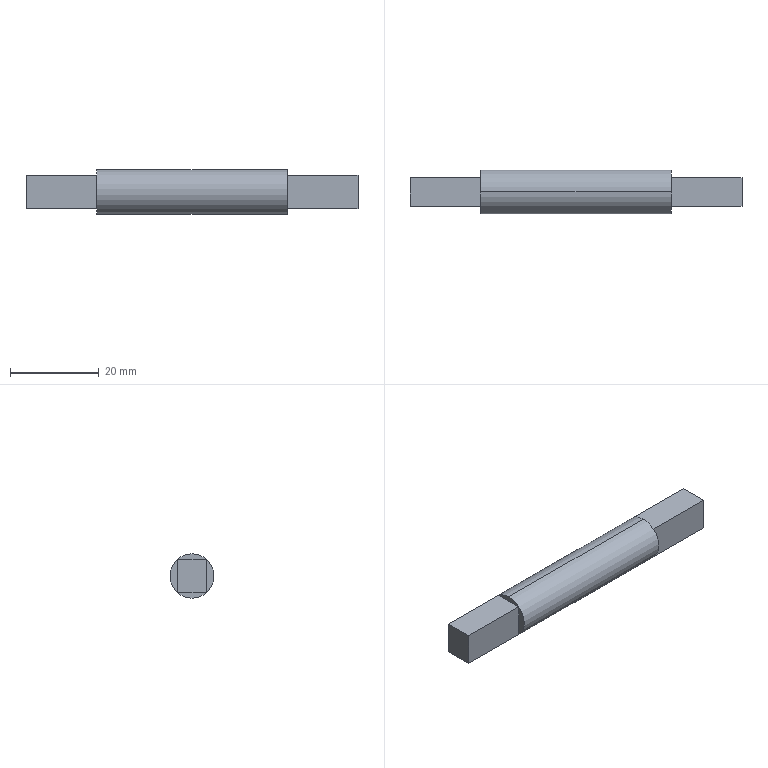Component | SolidWorks | CHEN123-AA-36-1 | 1 solid | 20 faces | box 75 x 10 x 10 mm | volume 4953 mm3 | plane 18 | cylinder 2 | commonest cylinder face diameters 10 x2
build123d program:
from build123d import *

# Parameters (mm, degrees)
SKETCH1_R           = 5
BOSS_EXTRUDE1_DEPTH = 75
SKETCH3_R           = 7.619
SKETCH3_W           = 7.664
SKETCH3_H           = 6.424
CUT_EXTRUDE2_DEPTH  = 16
SKETCH4_R           = 7.619
SKETCH4_W           = 7.664
SKETCH4_H           = 6.424
CUT_EXTRUDE3_DEPTH  = 16


with BuildPart() as part:
    # Sketch1 → Boss-Extrude1 (new body)
    with BuildSketch(Plane.XY):
        Circle(SKETCH1_R)
    extrude(amount=BOSS_EXTRUDE1_DEPTH)

    # Sketch3 → Cut-Extrude2 (cut)
    with BuildSketch(Plane.XY.offset(75)):
        Circle(SKETCH3_R)
        Rectangle(SKETCH3_W, SKETCH3_H, mode=Mode.SUBTRACT)
    extrude(amount=-CUT_EXTRUDE2_DEPTH, mode=Mode.SUBTRACT)

    # Sketch4 → Cut-Extrude3 (cut)
    with BuildSketch(Plane(origin=(0, 0, 0), x_dir=(-1, 0, 0), z_dir=(0, 0, -1))):
        Circle(SKETCH4_R)
        Rectangle(SKETCH4_W, SKETCH4_H, mode=Mode.SUBTRACT)
    extrude(amount=-CUT_EXTRUDE3_DEPTH, mode=Mode.SUBTRACT)


solid = part.part

# Placed as in the assembly
solid = solid.moved(Location((-37.501, -45.999, -172), (0, 90, 0)))
STEP:
#1=COLOUR_RGB('',0.7922,0.8196,0.9333);
#2=FILL_AREA_STYLE_COLOUR('',#1);
#3=FILL_AREA_STYLE('',(#2));
#4=SURFACE_STYLE_FILL_AREA(#3);
#5=SURFACE_SIDE_STYLE('',(#4));
#6=SURFACE_STYLE_USAGE(.BOTH.,#5);
#7=PRESENTATION_STYLE_ASSIGNMENT((#6));
#8=CARTESIAN_POINT('',(-0.8465,-1.811,-6.575));
#9=VERTEX_POINT('',#8);
#10=CARTESIAN_POINT('',(-0.8465,-1.685,-6.621));
#11=VERTEX_POINT('',#10);
#12=CARTESIAN_POINT('',(-0.8465,-1.811,-6.772));
#13=DIRECTION('',(-1.,0.,0.));
#14=DIRECTION('',(0.,0.,1.));
#15=AXIS2_PLACEMENT_3D('',#12,#13,#14);
#16=CIRCLE('',#15,0.1969);
#17=EDGE_CURVE('',#9,#11,#16,.T.);
#18=ORIENTED_EDGE('',*,*,#17,.F.);
#19=CARTESIAN_POINT('',(0.8464,-1.811,-6.575));
#20=VERTEX_POINT('',#19);
#21=CARTESIAN_POINT('',(-1.476,-1.811,-6.575));
#22=DIRECTION('',(1.,-0.,0.));
#23=VECTOR('',#22,39.37);
#24=LINE('',#21,#23);
#25=EDGE_CURVE('',#9,#20,#24,.T.);
#26=ORIENTED_EDGE('',*,*,#25,.T.);
#27=CARTESIAN_POINT('',(0.8464,-1.685,-6.621));
#28=VERTEX_POINT('',#27);
#29=CARTESIAN_POINT('',(0.8464,-1.811,-6.772));
#30=DIRECTION('',(1.,-0.,0.));
#31=DIRECTION('',(0.,0.,-1.));
#32=AXIS2_PLACEMENT_3D('',#29,#30,#31);
#33=CIRCLE('',#32,0.1969);
#34=EDGE_CURVE('',#28,#20,#33,.T.);
#35=ORIENTED_EDGE('',*,*,#34,.F.);
#36=CARTESIAN_POINT('',(0.8464,-1.685,-6.923));
#37=VERTEX_POINT('',#36);
#38=CARTESIAN_POINT('',(0.8464,-1.811,-6.772));
#39=DIRECTION('',(1.,-0.,0.));
#40=DIRECTION('',(0.,0.,-1.));
#41=AXIS2_PLACEMENT_3D('',#38,#39,#40);
#42=CIRCLE('',#41,0.1969);
#43=EDGE_CURVE('',#37,#28,#42,.T.);
#44=ORIENTED_EDGE('',*,*,#43,.F.);
#45=CARTESIAN_POINT('',(0.8464,-1.811,-6.969));
#46=VERTEX_POINT('',#45);
#47=CARTESIAN_POINT('',(0.8464,-1.811,-6.772));
#48=DIRECTION('',(1.,-0.,0.));
#49=DIRECTION('',(0.,0.,-1.));
#50=AXIS2_PLACEMENT_3D('',#47,#48,#49);
#51=CIRCLE('',#50,0.1969);
#52=EDGE_CURVE('',#46,#37,#51,.T.);
#53=ORIENTED_EDGE('',*,*,#52,.F.);
#54=CARTESIAN_POINT('',(-0.8465,-1.811,-6.969));
#55=VERTEX_POINT('',#54);
#56=CARTESIAN_POINT('',(-1.476,-1.811,-6.969));
#57=DIRECTION('',(1.,-0.,0.));
#58=VECTOR('',#57,39.37);
#59=LINE('',#56,#58);
#60=EDGE_CURVE('',#55,#46,#59,.T.);
#61=ORIENTED_EDGE('',*,*,#60,.F.);
#62=CARTESIAN_POINT('',(-0.8465,-1.685,-6.923));
#63=VERTEX_POINT('',#62);
#64=CARTESIAN_POINT('',(-0.8465,-1.811,-6.772));
#65=DIRECTION('',(-1.,0.,0.));
#66=DIRECTION('',(0.,0.,1.));
#67=AXIS2_PLACEMENT_3D('',#64,#65,#66);
#68=CIRCLE('',#67,0.1969);
#69=EDGE_CURVE('',#63,#55,#68,.T.);
#70=ORIENTED_EDGE('',*,*,#69,.F.);
#71=CARTESIAN_POINT('',(-0.8465,-1.811,-6.772));
#72=DIRECTION('',(-1.,0.,0.));
#73=DIRECTION('',(0.,0.,1.));
#74=AXIS2_PLACEMENT_3D('',#71,#72,#73);
#75=CIRCLE('',#74,0.1969);
#76=EDGE_CURVE('',#11,#63,#75,.T.);
#77=ORIENTED_EDGE('',*,*,#76,.F.);
#78=EDGE_LOOP('',(#18,#26,#35,#44,#53,#61,#70,#77));
#79=FACE_OUTER_BOUND('',#78,.T.);
#80=CARTESIAN_POINT('',(-1.476,-1.811,-6.772));
#81=DIRECTION('',(1.,-0.,0.));
#82=DIRECTION('',(0.,0.,-1.));
#83=AXIS2_PLACEMENT_3D('',#80,#81,#82);
#84=CYLINDRICAL_SURFACE('',#83,0.1969);
#85=ADVANCED_FACE('',(#79),#84,.T.);
#86=ORIENTED_EDGE('',*,*,#25,.F.);
#87=CARTESIAN_POINT('',(-0.8465,-1.937,-6.621));
#88=VERTEX_POINT('',#87);
#89=CARTESIAN_POINT('',(-0.8465,-1.811,-6.772));
#90=DIRECTION('',(-1.,0.,0.));
#91=DIRECTION('',(0.,0.,1.));
#92=AXIS2_PLACEMENT_3D('',#89,#90,#91);
#93=CIRCLE('',#92,0.1969);
#94=EDGE_CURVE('',#88,#9,#93,.T.);
#95=ORIENTED_EDGE('',*,*,#94,.F.);
#96=CARTESIAN_POINT('',(-0.8465,-1.937,-6.923));
#97=VERTEX_POINT('',#96);
#98=CARTESIAN_POINT('',(-0.8465,-1.811,-6.772));
#99=DIRECTION('',(-1.,0.,0.));
#100=DIRECTION('',(0.,0.,1.));
#101=AXIS2_PLACEMENT_3D('',#98,#99,#100);
#102=CIRCLE('',#101,0.1969);
#103=EDGE_CURVE('',#97,#88,#102,.T.);
#104=ORIENTED_EDGE('',*,*,#103,.F.);
#105=CARTESIAN_POINT('',(-0.8465,-1.811,-6.772));
#106=DIRECTION('',(-1.,0.,0.));
#107=DIRECTION('',(0.,0.,1.));
#108=AXIS2_PLACEMENT_3D('',#105,#106,#107);
#109=CIRCLE('',#108,0.1969);
#110=EDGE_CURVE('',#55,#97,#109,.T.);
#111=ORIENTED_EDGE('',*,*,#110,.F.);
#112=ORIENTED_EDGE('',*,*,#60,.T.);
#113=CARTESIAN_POINT('',(0.8464,-1.937,-6.923));
#114=VERTEX_POINT('',#113);
#115=CARTESIAN_POINT('',(0.8464,-1.811,-6.772));
#116=DIRECTION('',(1.,-0.,0.));
#117=DIRECTION('',(0.,0.,-1.));
#118=AXIS2_PLACEMENT_3D('',#115,#116,#117);
#119=CIRCLE('',#118,0.1969);
#120=EDGE_CURVE('',#114,#46,#119,.T.);
#121=ORIENTED_EDGE('',*,*,#120,.F.);
#122=CARTESIAN_POINT('',(0.8464,-1.937,-6.621));
#123=VERTEX_POINT('',#122);
#124=CARTESIAN_POINT('',(0.8464,-1.811,-6.772));
#125=DIRECTION('',(1.,-0.,0.));
#126=DIRECTION('',(0.,0.,-1.));
#127=AXIS2_PLACEMENT_3D('',#124,#125,#126);
#128=CIRCLE('',#127,0.1969);
#129=EDGE_CURVE('',#123,#114,#128,.T.);
#130=ORIENTED_EDGE('',*,*,#129,.F.);
#131=CARTESIAN_POINT('',(0.8464,-1.811,-6.772));
#132=DIRECTION('',(1.,-0.,0.));
#133=DIRECTION('',(0.,0.,-1.));
#134=AXIS2_PLACEMENT_3D('',#131,#132,#133);
#135=CIRCLE('',#134,0.1969);
#136=EDGE_CURVE('',#20,#123,#135,.T.);
#137=ORIENTED_EDGE('',*,*,#136,.F.);
#138=EDGE_LOOP('',(#86,#95,#104,#111,#112,#121,#130,#137));
#139=FACE_OUTER_BOUND('',#138,.T.);
#140=CARTESIAN_POINT('',(-1.476,-1.811,-6.772));
#141=DIRECTION('',(1.,-0.,0.));
#142=DIRECTION('',(0.,0.,-1.));
#143=AXIS2_PLACEMENT_3D('',#140,#141,#142);
#144=CYLINDRICAL_SURFACE('',#143,0.1969);
#145=ADVANCED_FACE('',(#139),#144,.T.);
#146=ORIENTED_EDGE('',*,*,#76,.T.);
#147=CARTESIAN_POINT('',(-0.8465,-1.685,-6.923));
#148=DIRECTION('',(-0.,-0.,-1.));
#149=VECTOR('',#148,39.37);
#150=LINE('',#147,#149);
#151=EDGE_CURVE('',#11,#63,#150,.T.);
#152=ORIENTED_EDGE('',*,*,#151,.F.);
#153=EDGE_LOOP('',(#146,#152));
#154=FACE_OUTER_BOUND('',#153,.T.);
#155=CARTESIAN_POINT('',(-0.8465,-1.811,-6.772));
#156=DIRECTION('',(-1.,0.,0.));
#157=DIRECTION('',(0.,0.,1.));
#158=AXIS2_PLACEMENT_3D('',#155,#156,#157);
#159=PLANE('',#158);
#160=ADVANCED_FACE('',(#154),#159,.T.);
#161=ORIENTED_EDGE('',*,*,#69,.T.);
#162=ORIENTED_EDGE('',*,*,#110,.T.);
#163=CARTESIAN_POINT('',(-0.8465,-1.685,-6.923));
#164=DIRECTION('',(-0.,-1.,0.));
#165=VECTOR('',#164,39.37);
#166=LINE('',#163,#165);
#167=EDGE_CURVE('',#63,#97,#166,.T.);
#168=ORIENTED_EDGE('',*,*,#167,.F.);
#169=EDGE_LOOP('',(#161,#162,#168));
#170=FACE_OUTER_BOUND('',#169,.T.);
#171=CARTESIAN_POINT('',(-0.8465,-1.811,-6.772));
#172=DIRECTION('',(-1.,0.,0.));
#173=DIRECTION('',(0.,0.,1.));
#174=AXIS2_PLACEMENT_3D('',#171,#172,#173);
#175=PLANE('',#174);
#176=ADVANCED_FACE('',(#170),#175,.T.);
#177=ORIENTED_EDGE('',*,*,#103,.T.);
#178=CARTESIAN_POINT('',(-0.8465,-1.937,-6.923));
#179=DIRECTION('',(0.,0.,1.));
#180=VECTOR('',#179,39.37);
#181=LINE('',#178,#180);
#182=EDGE_CURVE('',#97,#88,#181,.T.);
#183=ORIENTED_EDGE('',*,*,#182,.F.);
#184=EDGE_LOOP('',(#177,#183));
#185=FACE_OUTER_BOUND('',#184,.T.);
#186=CARTESIAN_POINT('',(-0.8465,-1.811,-6.772));
#187=DIRECTION('',(-1.,0.,0.));
#188=DIRECTION('',(0.,0.,1.));
#189=AXIS2_PLACEMENT_3D('',#186,#187,#188);
#190=PLANE('',#189);
#191=ADVANCED_FACE('',(#185),#190,.T.);
#192=ORIENTED_EDGE('',*,*,#94,.T.);
#193=ORIENTED_EDGE('',*,*,#17,.T.);
#194=CARTESIAN_POINT('',(-0.8465,-1.685,-6.621));
#195=DIRECTION('',(0.,1.,-0.));
#196=VECTOR('',#195,39.37);
#197=LINE('',#194,#196);
#198=EDGE_CURVE('',#88,#11,#197,.T.);
#199=ORIENTED_EDGE('',*,*,#198,.F.);
#200=EDGE_LOOP('',(#192,#193,#199));
#201=FACE_OUTER_BOUND('',#200,.T.);
#202=CARTESIAN_POINT('',(-0.8465,-1.811,-6.772));
#203=DIRECTION('',(-1.,0.,0.));
#204=DIRECTION('',(0.,0.,1.));
#205=AXIS2_PLACEMENT_3D('',#202,#203,#204);
#206=PLANE('',#205);
#207=ADVANCED_FACE('',(#201),#206,.T.);
#208=CARTESIAN_POINT('',(-1.476,-1.937,-6.621));
#209=VERTEX_POINT('',#208);
#210=CARTESIAN_POINT('',(-1.476,-1.685,-6.621));
#211=VERTEX_POINT('',#210);
#212=CARTESIAN_POINT('',(-1.476,-1.685,-6.621));
#213=DIRECTION('',(0.,1.,-0.));
#214=VECTOR('',#213,39.37);
#215=LINE('',#212,#214);
#216=EDGE_CURVE('',#209,#211,#215,.T.);
#217=ORIENTED_EDGE('',*,*,#216,.F.);
#218=CARTESIAN_POINT('',(-0.8465,-1.937,-6.621));
#219=DIRECTION('',(-1.,0.,0.));
#220=VECTOR('',#219,39.37);
#221=LINE('',#218,#220);
#222=EDGE_CURVE('',#88,#209,#221,.T.);
#223=ORIENTED_EDGE('',*,*,#222,.F.);
#224=ORIENTED_EDGE('',*,*,#198,.T.);
#225=CARTESIAN_POINT('',(-0.8465,-1.685,-6.621));
#226=DIRECTION('',(-1.,0.,0.));
#227=VECTOR('',#226,39.37);
#228=LINE('',#225,#227);
#229=EDGE_CURVE('',#11,#211,#228,.T.);
#230=ORIENTED_EDGE('',*,*,#229,.T.);
#231=EDGE_LOOP('',(#217,#223,#224,#230));
#232=FACE_OUTER_BOUND('',#231,.T.);
#233=CARTESIAN_POINT('',(-0.8465,-1.685,-6.621));
#234=DIRECTION('',(0.,0.,1.));
#235=DIRECTION('',(1.,-0.,0.));
#236=AXIS2_PLACEMENT_3D('',#233,#234,#235);
#237=PLANE('',#236);
#238=ADVANCED_FACE('',(#232),#237,.T.);
#239=CARTESIAN_POINT('',(-1.476,-1.937,-6.923));
#240=VERTEX_POINT('',#239);
#241=CARTESIAN_POINT('',(-1.476,-1.937,-6.923));
#242=DIRECTION('',(0.,0.,1.));
#243=VECTOR('',#242,39.37);
#244=LINE('',#241,#243);
#245=EDGE_CURVE('',#240,#209,#244,.T.);
#246=ORIENTED_EDGE('',*,*,#245,.F.);
#247=CARTESIAN_POINT('',(-0.8465,-1.937,-6.923));
#248=DIRECTION('',(-1.,0.,0.));
#249=VECTOR('',#248,39.37);
#250=LINE('',#247,#249);
#251=EDGE_CURVE('',#97,#240,#250,.T.);
#252=ORIENTED_EDGE('',*,*,#251,.F.);
#253=ORIENTED_EDGE('',*,*,#182,.T.);
#254=ORIENTED_EDGE('',*,*,#222,.T.);
#255=EDGE_LOOP('',(#246,#252,#253,#254));
#256=FACE_OUTER_BOUND('',#255,.T.);
#257=CARTESIAN_POINT('',(-0.8465,-1.937,-6.923));
#258=DIRECTION('',(-0.,-1.,0.));
#259=DIRECTION('',(1.,-0.,0.));
#260=AXIS2_PLACEMENT_3D('',#257,#258,#259);
#261=PLANE('',#260);
#262=ADVANCED_FACE('',(#256),#261,.T.);
#263=CARTESIAN_POINT('',(-1.476,-1.685,-6.923));
#264=VERTEX_POINT('',#263);
#265=CARTESIAN_POINT('',(-1.476,-1.685,-6.923));
#266=DIRECTION('',(-0.,-1.,0.));
#267=VECTOR('',#266,39.37);
#268=LINE('',#265,#267);
#269=EDGE_CURVE('',#264,#240,#268,.T.);
#270=ORIENTED_EDGE('',*,*,#269,.F.);
#271=CARTESIAN_POINT('',(-0.8465,-1.685,-6.923));
#272=DIRECTION('',(-1.,0.,0.));
#273=VECTOR('',#272,39.37);
#274=LINE('',#271,#273);
#275=EDGE_CURVE('',#63,#264,#274,.T.);
#276=ORIENTED_EDGE('',*,*,#275,.F.);
#277=ORIENTED_EDGE('',*,*,#167,.T.);
#278=ORIENTED_EDGE('',*,*,#251,.T.);
#279=EDGE_LOOP('',(#270,#276,#277,#278));
#280=FACE_OUTER_BOUND('',#279,.T.);
#281=CARTESIAN_POINT('',(-0.8465,-1.685,-6.923));
#282=DIRECTION('',(-0.,-0.,-1.));
#283=DIRECTION('',(-1.,0.,0.));
#284=AXIS2_PLACEMENT_3D('',#281,#282,#283);
#285=PLANE('',#284);
#286=ADVANCED_FACE('',(#280),#285,.T.);
#287=CARTESIAN_POINT('',(-1.476,-1.685,-6.923));
#288=DIRECTION('',(-0.,-0.,-1.));
#289=VECTOR('',#288,39.37);
#290=LINE('',#287,#289);
#291=EDGE_CURVE('',#211,#264,#290,.T.);
#292=ORIENTED_EDGE('',*,*,#291,.F.);
#293=ORIENTED_EDGE('',*,*,#229,.F.);
#294=ORIENTED_EDGE('',*,*,#151,.T.);
#295=ORIENTED_EDGE('',*,*,#275,.T.);
#296=EDGE_LOOP('',(#292,#293,#294,#295));
#297=FACE_OUTER_BOUND('',#296,.T.);
#298=CARTESIAN_POINT('',(-0.8465,-1.685,-6.923));
#299=DIRECTION('',(0.,1.,-0.));
#300=DIRECTION('',(-1.,0.,0.));
#301=AXIS2_PLACEMENT_3D('',#298,#299,#300);
#302=PLANE('',#301);
#303=ADVANCED_FACE('',(#297),#302,.T.);
#304=ORIENTED_EDGE('',*,*,#245,.T.);
#305=ORIENTED_EDGE('',*,*,#216,.T.);
#306=ORIENTED_EDGE('',*,*,#291,.T.);
#307=ORIENTED_EDGE('',*,*,#269,.T.);
#308=EDGE_LOOP('',(#304,#305,#306,#307));
#309=FACE_OUTER_BOUND('',#308,.T.);
#310=CARTESIAN_POINT('',(-1.476,-1.811,-6.772));
#311=DIRECTION('',(-1.,0.,0.));
#312=DIRECTION('',(0.,0.,1.));
#313=AXIS2_PLACEMENT_3D('',#310,#311,#312);
#314=PLANE('',#313);
#315=ADVANCED_FACE('',(#309),#314,.T.);
#316=ORIENTED_EDGE('',*,*,#43,.T.);
#317=CARTESIAN_POINT('',(0.8464,-1.685,-6.923));
#318=DIRECTION('',(0.,0.,1.));
#319=VECTOR('',#318,39.37);
#320=LINE('',#317,#319);
#321=EDGE_CURVE('',#37,#28,#320,.T.);
#322=ORIENTED_EDGE('',*,*,#321,.F.);
#323=EDGE_LOOP('',(#316,#322));
#324=FACE_OUTER_BOUND('',#323,.T.);
#325=CARTESIAN_POINT('',(0.8464,-1.811,-6.772));
#326=DIRECTION('',(1.,-0.,0.));
#327=DIRECTION('',(-0.,-0.,-1.));
#328=AXIS2_PLACEMENT_3D('',#325,#326,#327);
#329=PLANE('',#328);
#330=ADVANCED_FACE('',(#324),#329,.T.);
#331=ORIENTED_EDGE('',*,*,#34,.T.);
#332=ORIENTED_EDGE('',*,*,#136,.T.);
#333=CARTESIAN_POINT('',(0.8464,-1.685,-6.621));
#334=DIRECTION('',(-0.,-1.,0.));
#335=VECTOR('',#334,39.37);
#336=LINE('',#333,#335);
#337=EDGE_CURVE('',#28,#123,#336,.T.);
#338=ORIENTED_EDGE('',*,*,#337,.F.);
#339=EDGE_LOOP('',(#331,#332,#338));
#340=FACE_OUTER_BOUND('',#339,.T.);
#341=CARTESIAN_POINT('',(0.8464,-1.811,-6.772));
#342=DIRECTION('',(1.,-0.,0.));
#343=DIRECTION('',(-0.,-0.,-1.));
#344=AXIS2_PLACEMENT_3D('',#341,#342,#343);
#345=PLANE('',#344);
#346=ADVANCED_FACE('',(#340),#345,.T.);
#347=ORIENTED_EDGE('',*,*,#129,.T.);
#348=CARTESIAN_POINT('',(0.8464,-1.937,-6.621));
#349=DIRECTION('',(-0.,-0.,-1.));
#350=VECTOR('',#349,39.37);
#351=LINE('',#348,#350);
#352=EDGE_CURVE('',#123,#114,#351,.T.);
#353=ORIENTED_EDGE('',*,*,#352,.F.);
#354=EDGE_LOOP('',(#347,#353));
#355=FACE_OUTER_BOUND('',#354,.T.);
#356=CARTESIAN_POINT('',(0.8464,-1.811,-6.772));
#357=DIRECTION('',(1.,-0.,0.));
#358=DIRECTION('',(-0.,-0.,-1.));
#359=AXIS2_PLACEMENT_3D('',#356,#357,#358);
#360=PLANE('',#359);
#361=ADVANCED_FACE('',(#355),#360,.T.);
#362=ORIENTED_EDGE('',*,*,#120,.T.);
#363=ORIENTED_EDGE('',*,*,#52,.T.);
#364=CARTESIAN_POINT('',(0.8464,-1.937,-6.923));
#365=DIRECTION('',(0.,1.,-0.));
#366=VECTOR('',#365,39.37);
#367=LINE('',#364,#366);
#368=EDGE_CURVE('',#114,#37,#367,.T.);
#369=ORIENTED_EDGE('',*,*,#368,.F.);
#370=EDGE_LOOP('',(#362,#363,#369));
#371=FACE_OUTER_BOUND('',#370,.T.);
#372=CARTESIAN_POINT('',(0.8464,-1.811,-6.772));
#373=DIRECTION('',(1.,-0.,0.));
#374=DIRECTION('',(-0.,-0.,-1.));
#375=AXIS2_PLACEMENT_3D('',#372,#373,#374);
#376=PLANE('',#375);
#377=ADVANCED_FACE('',(#371),#376,.T.);
#378=CARTESIAN_POINT('',(1.476,-1.937,-6.923));
#379=VERTEX_POINT('',#378);
#380=CARTESIAN_POINT('',(1.476,-1.685,-6.923));
#381=VERTEX_POINT('',#380);
#382=CARTESIAN_POINT('',(1.476,-1.937,-6.923));
#383=DIRECTION('',(0.,1.,-0.));
#384=VECTOR('',#383,39.37);
#385=LINE('',#382,#384);
#386=EDGE_CURVE('',#379,#381,#385,.T.);
#387=ORIENTED_EDGE('',*,*,#386,.F.);
#388=CARTESIAN_POINT('',(0.8464,-1.937,-6.923));
#389=DIRECTION('',(1.,-0.,0.));
#390=VECTOR('',#389,39.37);
#391=LINE('',#388,#390);
#392=EDGE_CURVE('',#114,#379,#391,.T.);
#393=ORIENTED_EDGE('',*,*,#392,.F.);
#394=ORIENTED_EDGE('',*,*,#368,.T.);
#395=CARTESIAN_POINT('',(0.8464,-1.685,-6.923));
#396=DIRECTION('',(1.,-0.,0.));
#397=VECTOR('',#396,39.37);
#398=LINE('',#395,#397);
#399=EDGE_CURVE('',#37,#381,#398,.T.);
#400=ORIENTED_EDGE('',*,*,#399,.T.);
#401=EDGE_LOOP('',(#387,#393,#394,#400));
#402=FACE_OUTER_BOUND('',#401,.T.);
#403=CARTESIAN_POINT('',(0.8464,-1.937,-6.923));
#404=DIRECTION('',(-0.,-0.,-1.));
#405=DIRECTION('',(-1.,0.,0.));
#406=AXIS2_PLACEMENT_3D('',#403,#404,#405);
#407=PLANE('',#406);
#408=ADVANCED_FACE('',(#402),#407,.T.);
#409=CARTESIAN_POINT('',(1.476,-1.937,-6.621));
#410=VERTEX_POINT('',#409);
#411=CARTESIAN_POINT('',(1.476,-1.937,-6.621));
#412=DIRECTION('',(-0.,-0.,-1.));
#413=VECTOR('',#412,39.37);
#414=LINE('',#411,#413);
#415=EDGE_CURVE('',#410,#379,#414,.T.);
#416=ORIENTED_EDGE('',*,*,#415,.F.);
#417=CARTESIAN_POINT('',(0.8464,-1.937,-6.621));
#418=DIRECTION('',(1.,-0.,0.));
#419=VECTOR('',#418,39.37);
#420=LINE('',#417,#419);
#421=EDGE_CURVE('',#123,#410,#420,.T.);
#422=ORIENTED_EDGE('',*,*,#421,.F.);
#423=ORIENTED_EDGE('',*,*,#352,.T.);
#424=ORIENTED_EDGE('',*,*,#392,.T.);
#425=EDGE_LOOP('',(#416,#422,#423,#424));
#426=FACE_OUTER_BOUND('',#425,.T.);
#427=CARTESIAN_POINT('',(0.8464,-1.937,-6.621));
#428=DIRECTION('',(-0.,-1.,0.));
#429=DIRECTION('',(1.,-0.,0.));
#430=AXIS2_PLACEMENT_3D('',#427,#428,#429);
#431=PLANE('',#430);
#432=ADVANCED_FACE('',(#426),#431,.T.);
#433=CARTESIAN_POINT('',(1.476,-1.685,-6.621));
#434=VERTEX_POINT('',#433);
#435=CARTESIAN_POINT('',(1.476,-1.685,-6.621));
#436=DIRECTION('',(-0.,-1.,0.));
#437=VECTOR('',#436,39.37);
#438=LINE('',#435,#437);
#439=EDGE_CURVE('',#434,#410,#438,.T.);
#440=ORIENTED_EDGE('',*,*,#439,.F.);
#441=CARTESIAN_POINT('',(0.8464,-1.685,-6.621));
#442=DIRECTION('',(1.,-0.,0.));
#443=VECTOR('',#442,39.37);
#444=LINE('',#441,#443);
#445=EDGE_CURVE('',#28,#434,#444,.T.);
#446=ORIENTED_EDGE('',*,*,#445,.F.);
#447=ORIENTED_EDGE('',*,*,#337,.T.);
#448=ORIENTED_EDGE('',*,*,#421,.T.);
#449=EDGE_LOOP('',(#440,#446,#447,#448));
#450=FACE_OUTER_BOUND('',#449,.T.);
#451=CARTESIAN_POINT('',(0.8464,-1.685,-6.621));
#452=DIRECTION('',(0.,0.,1.));
#453=DIRECTION('',(1.,-0.,0.));
#454=AXIS2_PLACEMENT_3D('',#451,#452,#453);
#455=PLANE('',#454);
#456=ADVANCED_FACE('',(#450),#455,.T.);
#457=CARTESIAN_POINT('',(1.476,-1.685,-6.923));
#458=DIRECTION('',(0.,0.,1.));
#459=VECTOR('',#458,39.37);
#460=LINE('',#457,#459);
#461=EDGE_CURVE('',#381,#434,#460,.T.);
#462=ORIENTED_EDGE('',*,*,#461,.F.);
#463=ORIENTED_EDGE('',*,*,#399,.F.);
#464=ORIENTED_EDGE('',*,*,#321,.T.);
#465=ORIENTED_EDGE('',*,*,#445,.T.);
#466=EDGE_LOOP('',(#462,#463,#464,#465));
#467=FACE_OUTER_BOUND('',#466,.T.);
#468=CARTESIAN_POINT('',(0.8464,-1.685,-6.923));
#469=DIRECTION('',(0.,1.,-0.));
#470=DIRECTION('',(-1.,0.,0.));
#471=AXIS2_PLACEMENT_3D('',#468,#469,#470);
#472=PLANE('',#471);
#473=ADVANCED_FACE('',(#467),#472,.T.);
#474=ORIENTED_EDGE('',*,*,#386,.T.);
#475=ORIENTED_EDGE('',*,*,#461,.T.);
#476=ORIENTED_EDGE('',*,*,#439,.T.);
#477=ORIENTED_EDGE('',*,*,#415,.T.);
#478=EDGE_LOOP('',(#474,#475,#476,#477));
#479=FACE_OUTER_BOUND('',#478,.T.);
#480=CARTESIAN_POINT('',(1.476,-1.811,-6.772));
#481=DIRECTION('',(-1.,0.,0.));
#482=DIRECTION('',(0.,0.,1.));
#483=AXIS2_PLACEMENT_3D('',#480,#481,#482);
#484=PLANE('',#483);
#485=ADVANCED_FACE('',(#479),#484,.F.);
#486=CLOSED_SHELL('',(#85,#145,#160,#176,#191,#207,#238,#262,#286,#303,#315,#330,#346,#361,#377,#408,#432,#456,#473,#485));
#487=MANIFOLD_SOLID_BREP('',#486);
#488=STYLED_ITEM('',(#7),#487);
#489=PRESENTATION_LAYER_ASSIGNMENT('','',(#488));
#490=CARTESIAN_POINT('',(0.,0.,0.));
#491=DIRECTION('',(0.,0.,1.));
#492=DIRECTION('',(1.,0.,0.));
#493=AXIS2_PLACEMENT_3D('',#490,#491,#492);
#494=(LENGTH_UNIT()NAMED_UNIT(*)SI_UNIT($,.METRE.));
#495=LENGTH_MEASURE_WITH_UNIT(LENGTH_MEASURE(0.0254),#494);
#496=DIMENSIONAL_EXPONENTS(1.,0.,0.,0.,0.,0.,0.);
#497=(CONVERSION_BASED_UNIT('',#495)LENGTH_UNIT()NAMED_UNIT(#496));
#498=UNCERTAINTY_MEASURE_WITH_UNIT(LENGTH_MEASURE(0.00001),#497,'','');
#499=(NAMED_UNIT(*)PLANE_ANGLE_UNIT()SI_UNIT($,.RADIAN.));
#500=(NAMED_UNIT(*)SI_UNIT($,.STERADIAN.)SOLID_ANGLE_UNIT());
#501=(GEOMETRIC_REPRESENTATION_CONTEXT(3)GLOBAL_UNCERTAINTY_ASSIGNED_CONTEXT((#498))GLOBAL_UNIT_ASSIGNED_CONTEXT((#497,#499,#500))REPRESENTATION_CONTEXT('',''));
#502=ADVANCED_BREP_SHAPE_REPRESENTATION('',(#487,#493),#501);
#503=(LENGTH_UNIT()NAMED_UNIT(*)SI_UNIT($,.METRE.));
#504=LENGTH_MEASURE_WITH_UNIT(LENGTH_MEASURE(0.0254),#503);
#505=DIMENSIONAL_EXPONENTS(1.,0.,0.,0.,0.,0.,0.);
#506=(CONVERSION_BASED_UNIT('',#504)LENGTH_UNIT()NAMED_UNIT(#505));
#507=UNCERTAINTY_MEASURE_WITH_UNIT(LENGTH_MEASURE(0.00001),#506,'','');
#508=(NAMED_UNIT(*)PLANE_ANGLE_UNIT()SI_UNIT($,.RADIAN.));
#509=(NAMED_UNIT(*)SI_UNIT($,.STERADIAN.)SOLID_ANGLE_UNIT());
#510=(GEOMETRIC_REPRESENTATION_CONTEXT(3)GLOBAL_UNCERTAINTY_ASSIGNED_CONTEXT((#507))GLOBAL_UNIT_ASSIGNED_CONTEXT((#506,#508,#509))REPRESENTATION_CONTEXT('',''));
#511=MECHANICAL_DESIGN_GEOMETRIC_PRESENTATION_REPRESENTATION('',(#488),#510);